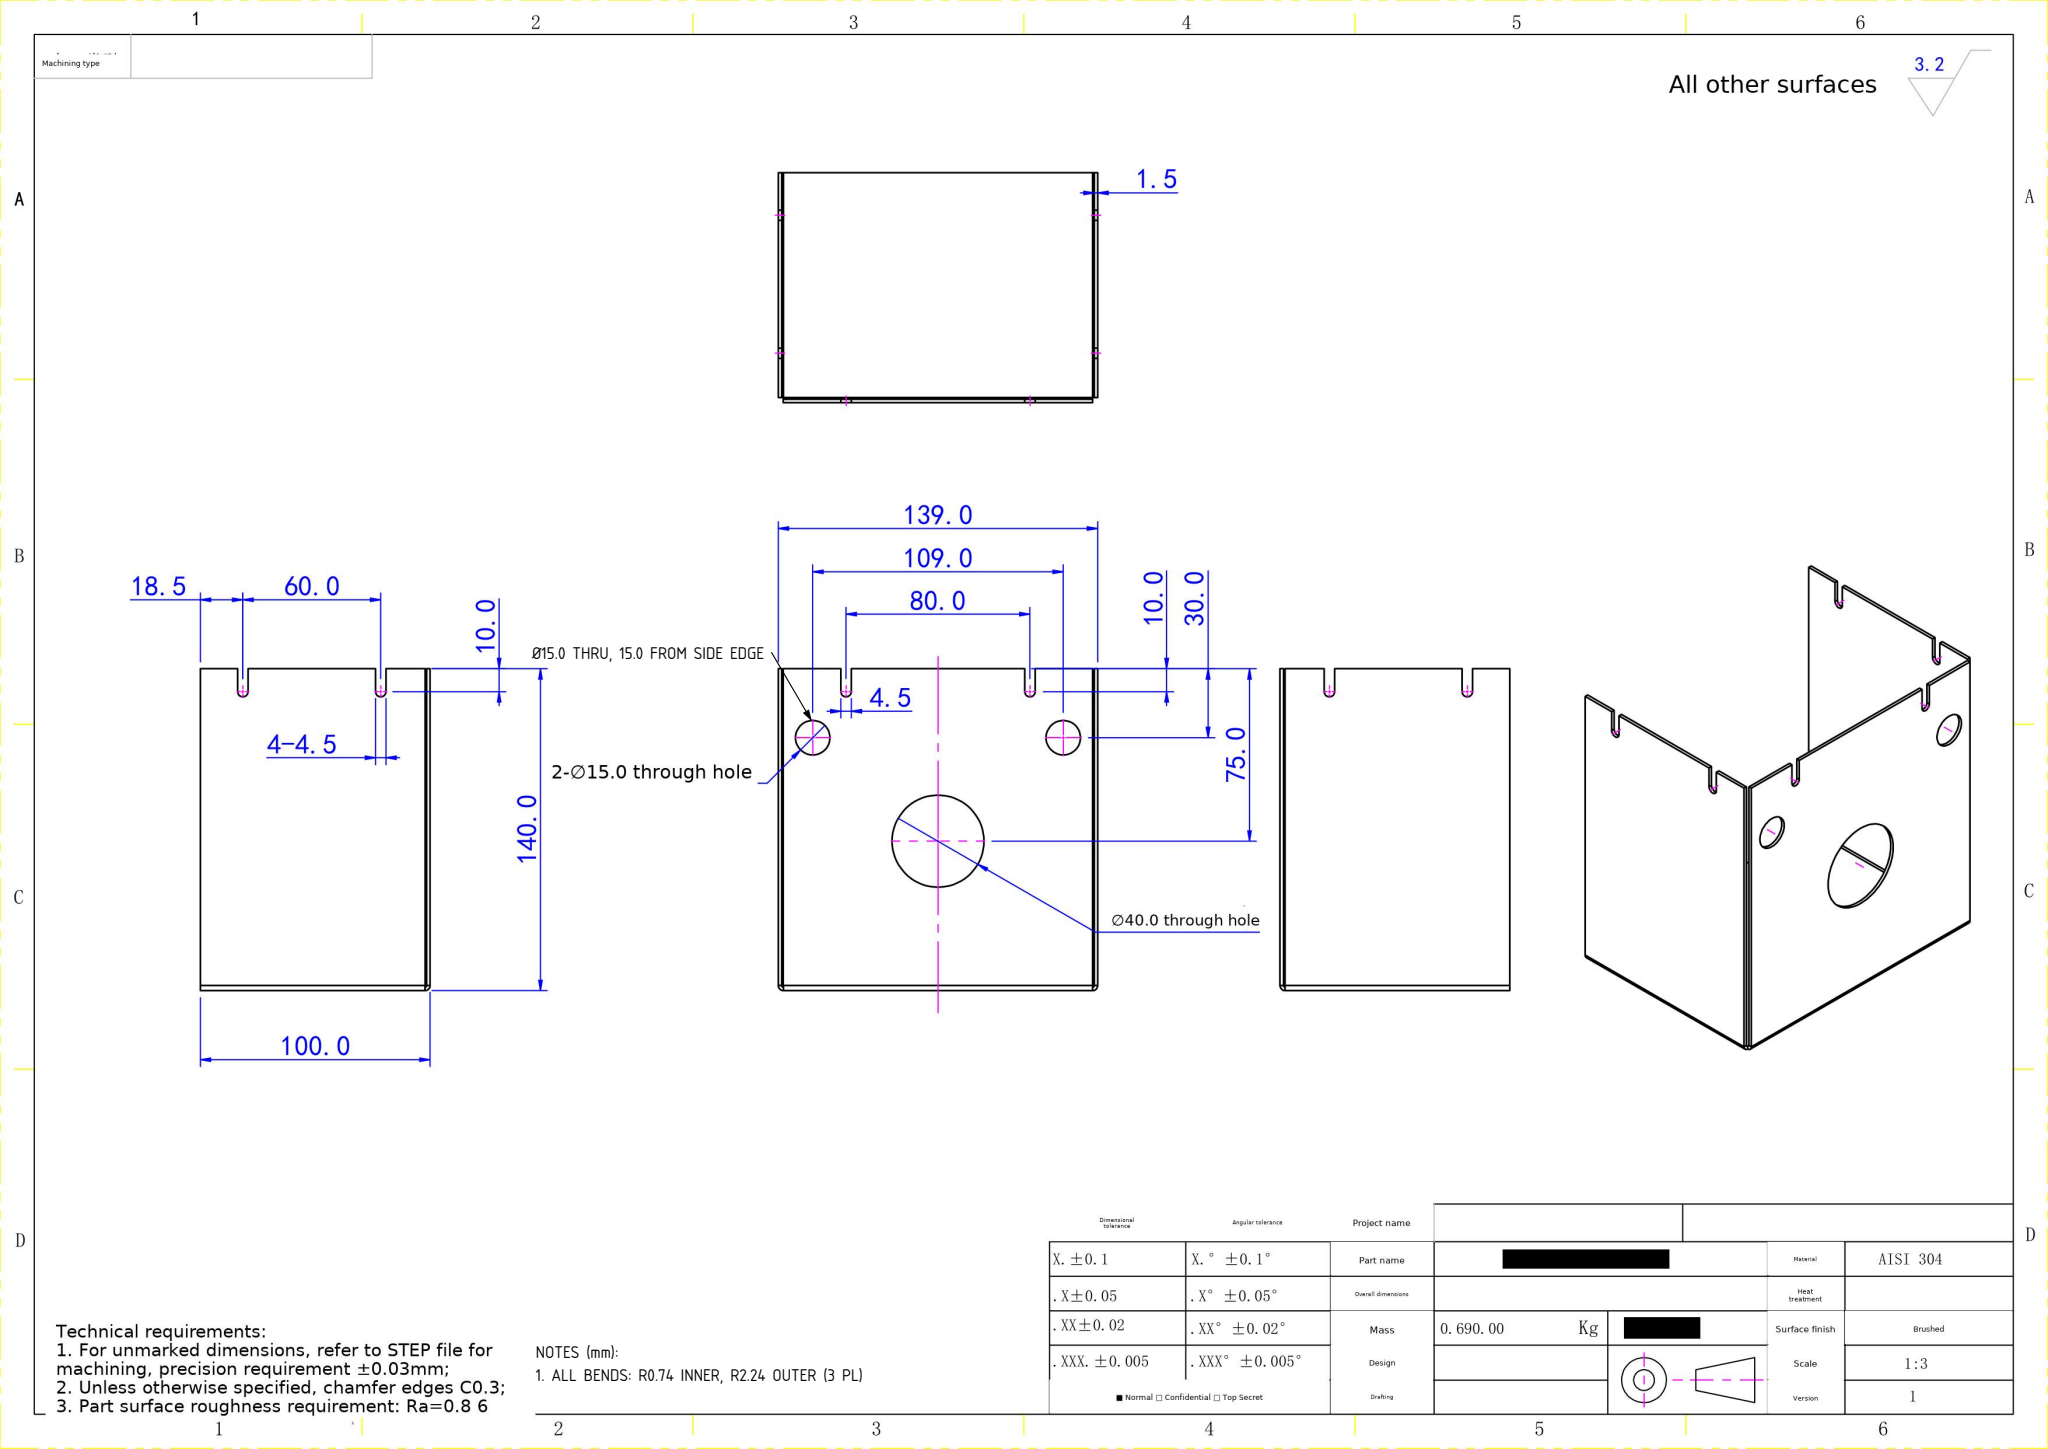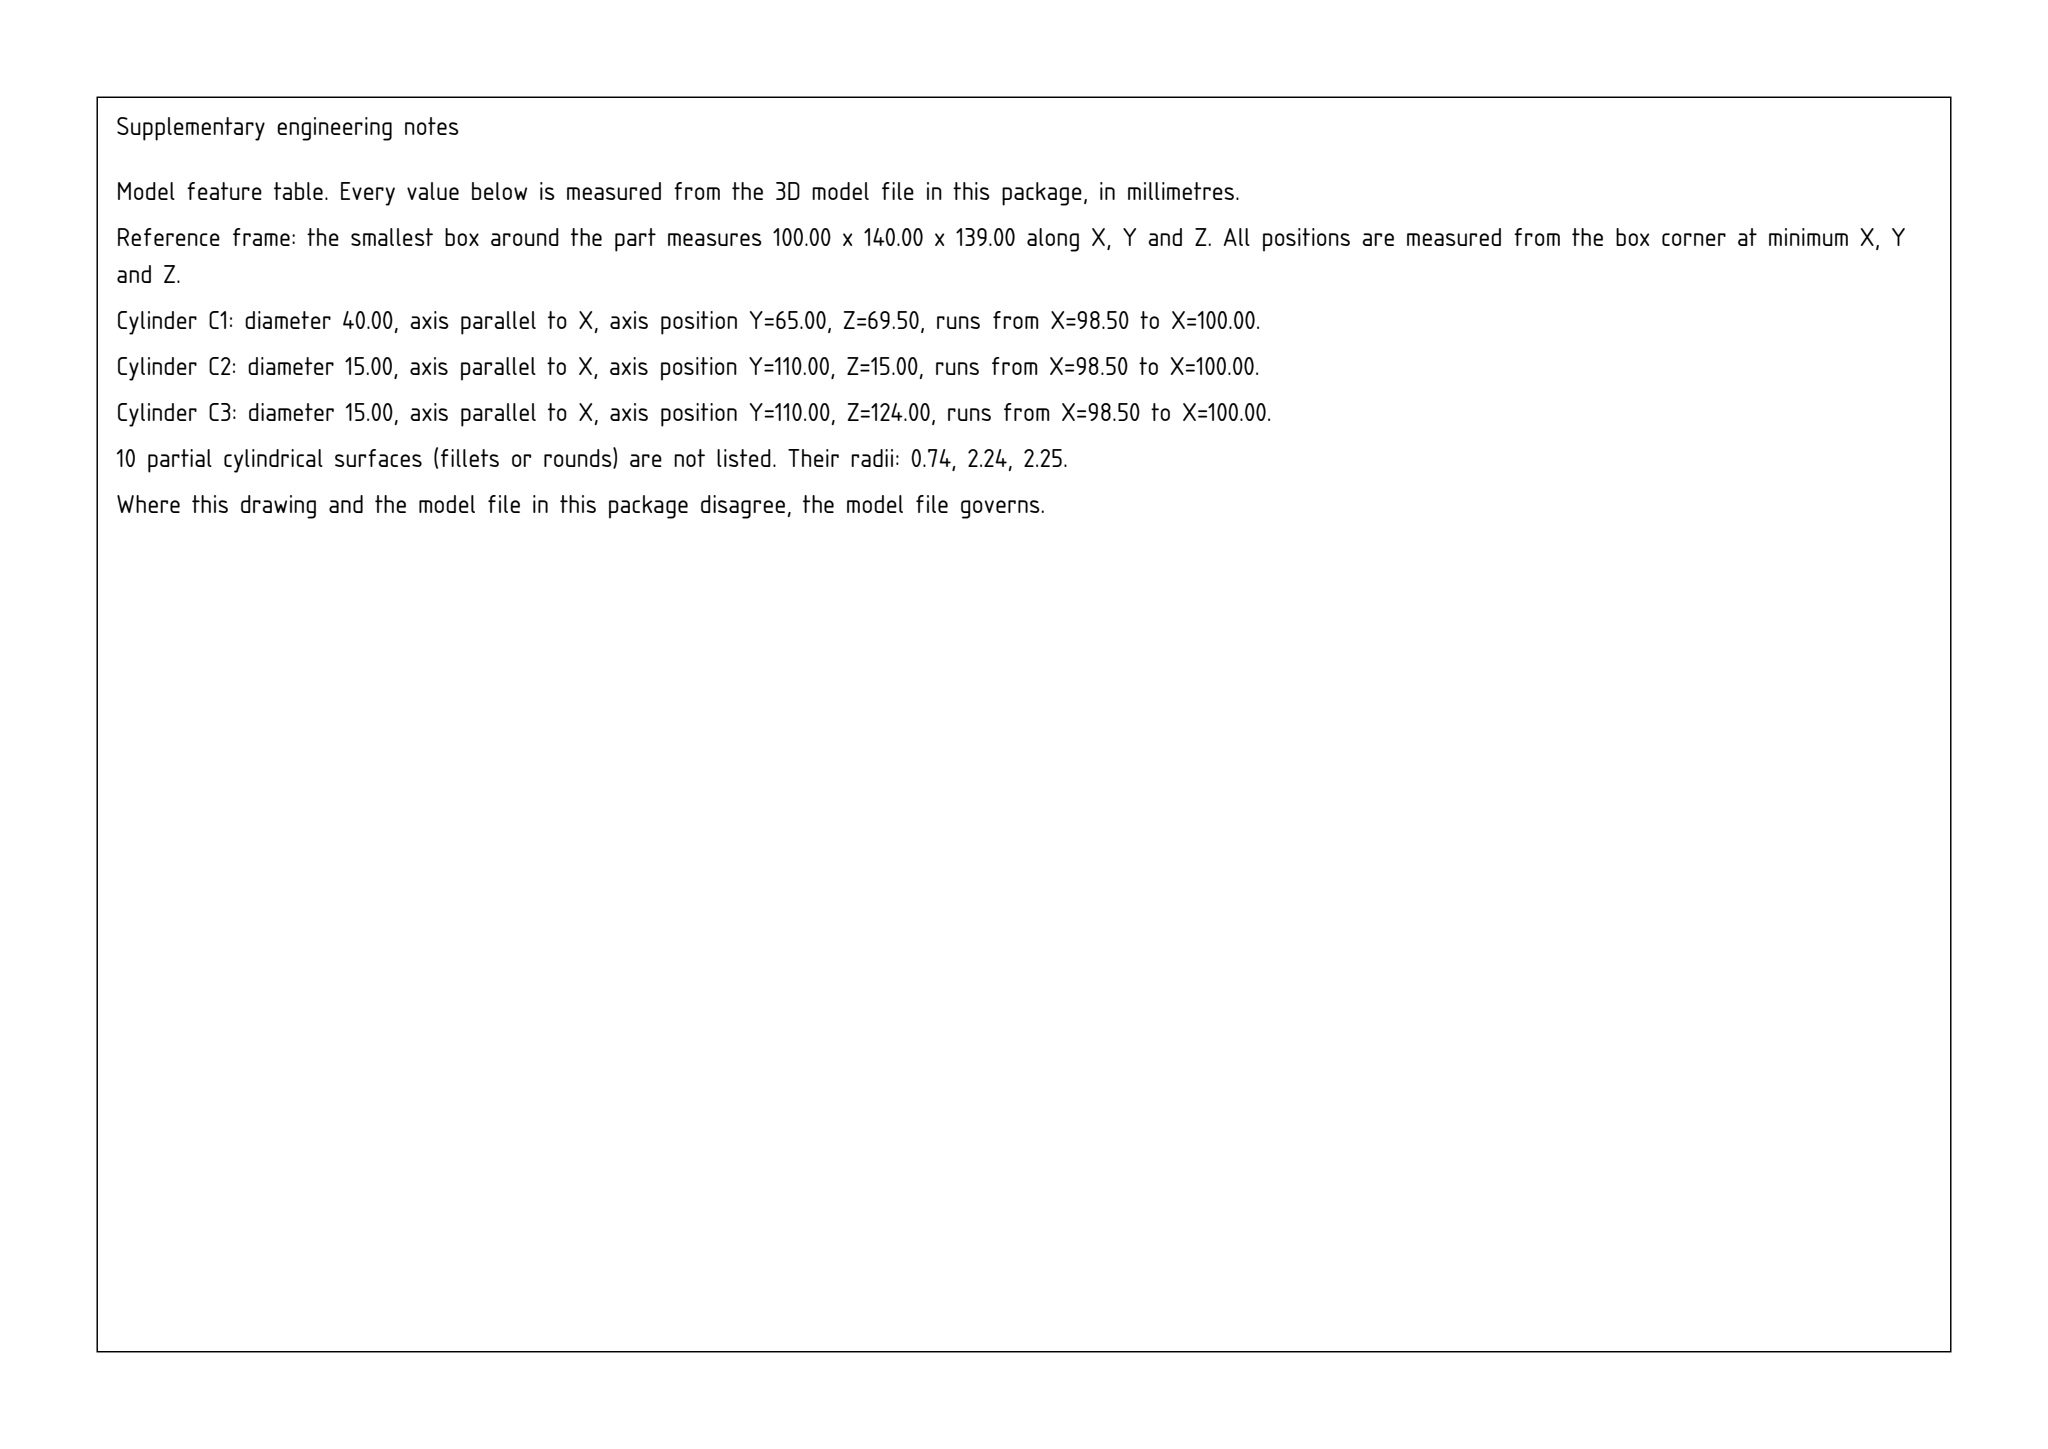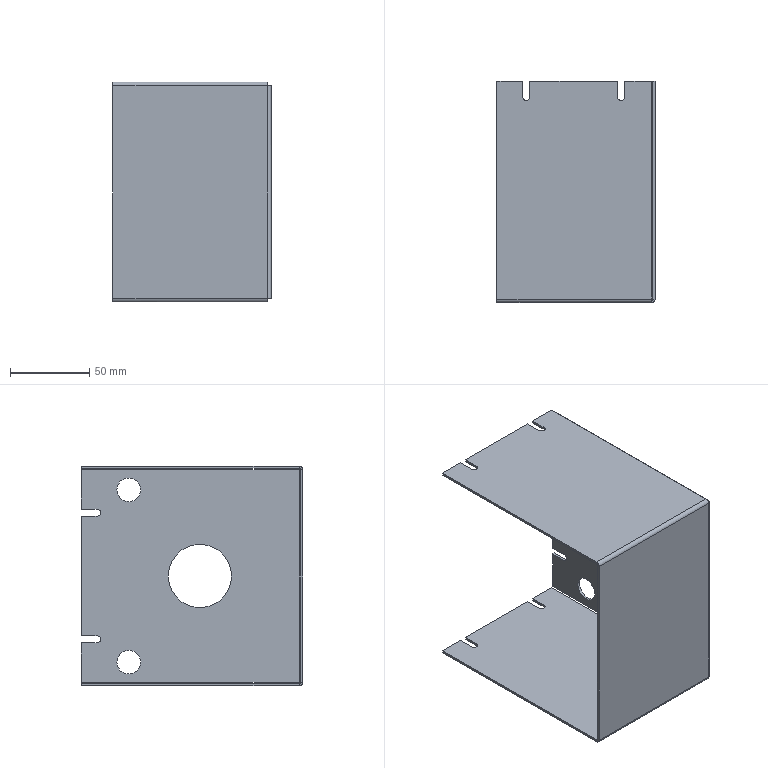Part | SolidWorks | mm | material AISI 304 | 1 solid | 60 faces | box 100 x 140 x 139 mm | volume 86221 mm3 | plane 38 | cylinder 18 | spline 4 | commonest cylinder face diameters 4.5 x6 15 x4 4.473 x3 1.473 x3 40 x2
Drawing notes:
2-Ø15.0 THRU: 15.0 FROM EACH SIDE EDGE, 109.0 BETWEEN CTRS | from the solid: Ø15.0 x-axis cyls at z=15.02 and z=124.02; wall z-extent 0.02 to 139.02 (139.0 wide)
ALL BENDS: R0.74 INNER, R2.24 OUTER (3 PL) | from the solid: Bend fillet cyls Ø1.473 (R0.74) and Ø4.473 (R2.24), 3 corners (2 x-axis, 1 z-axis)